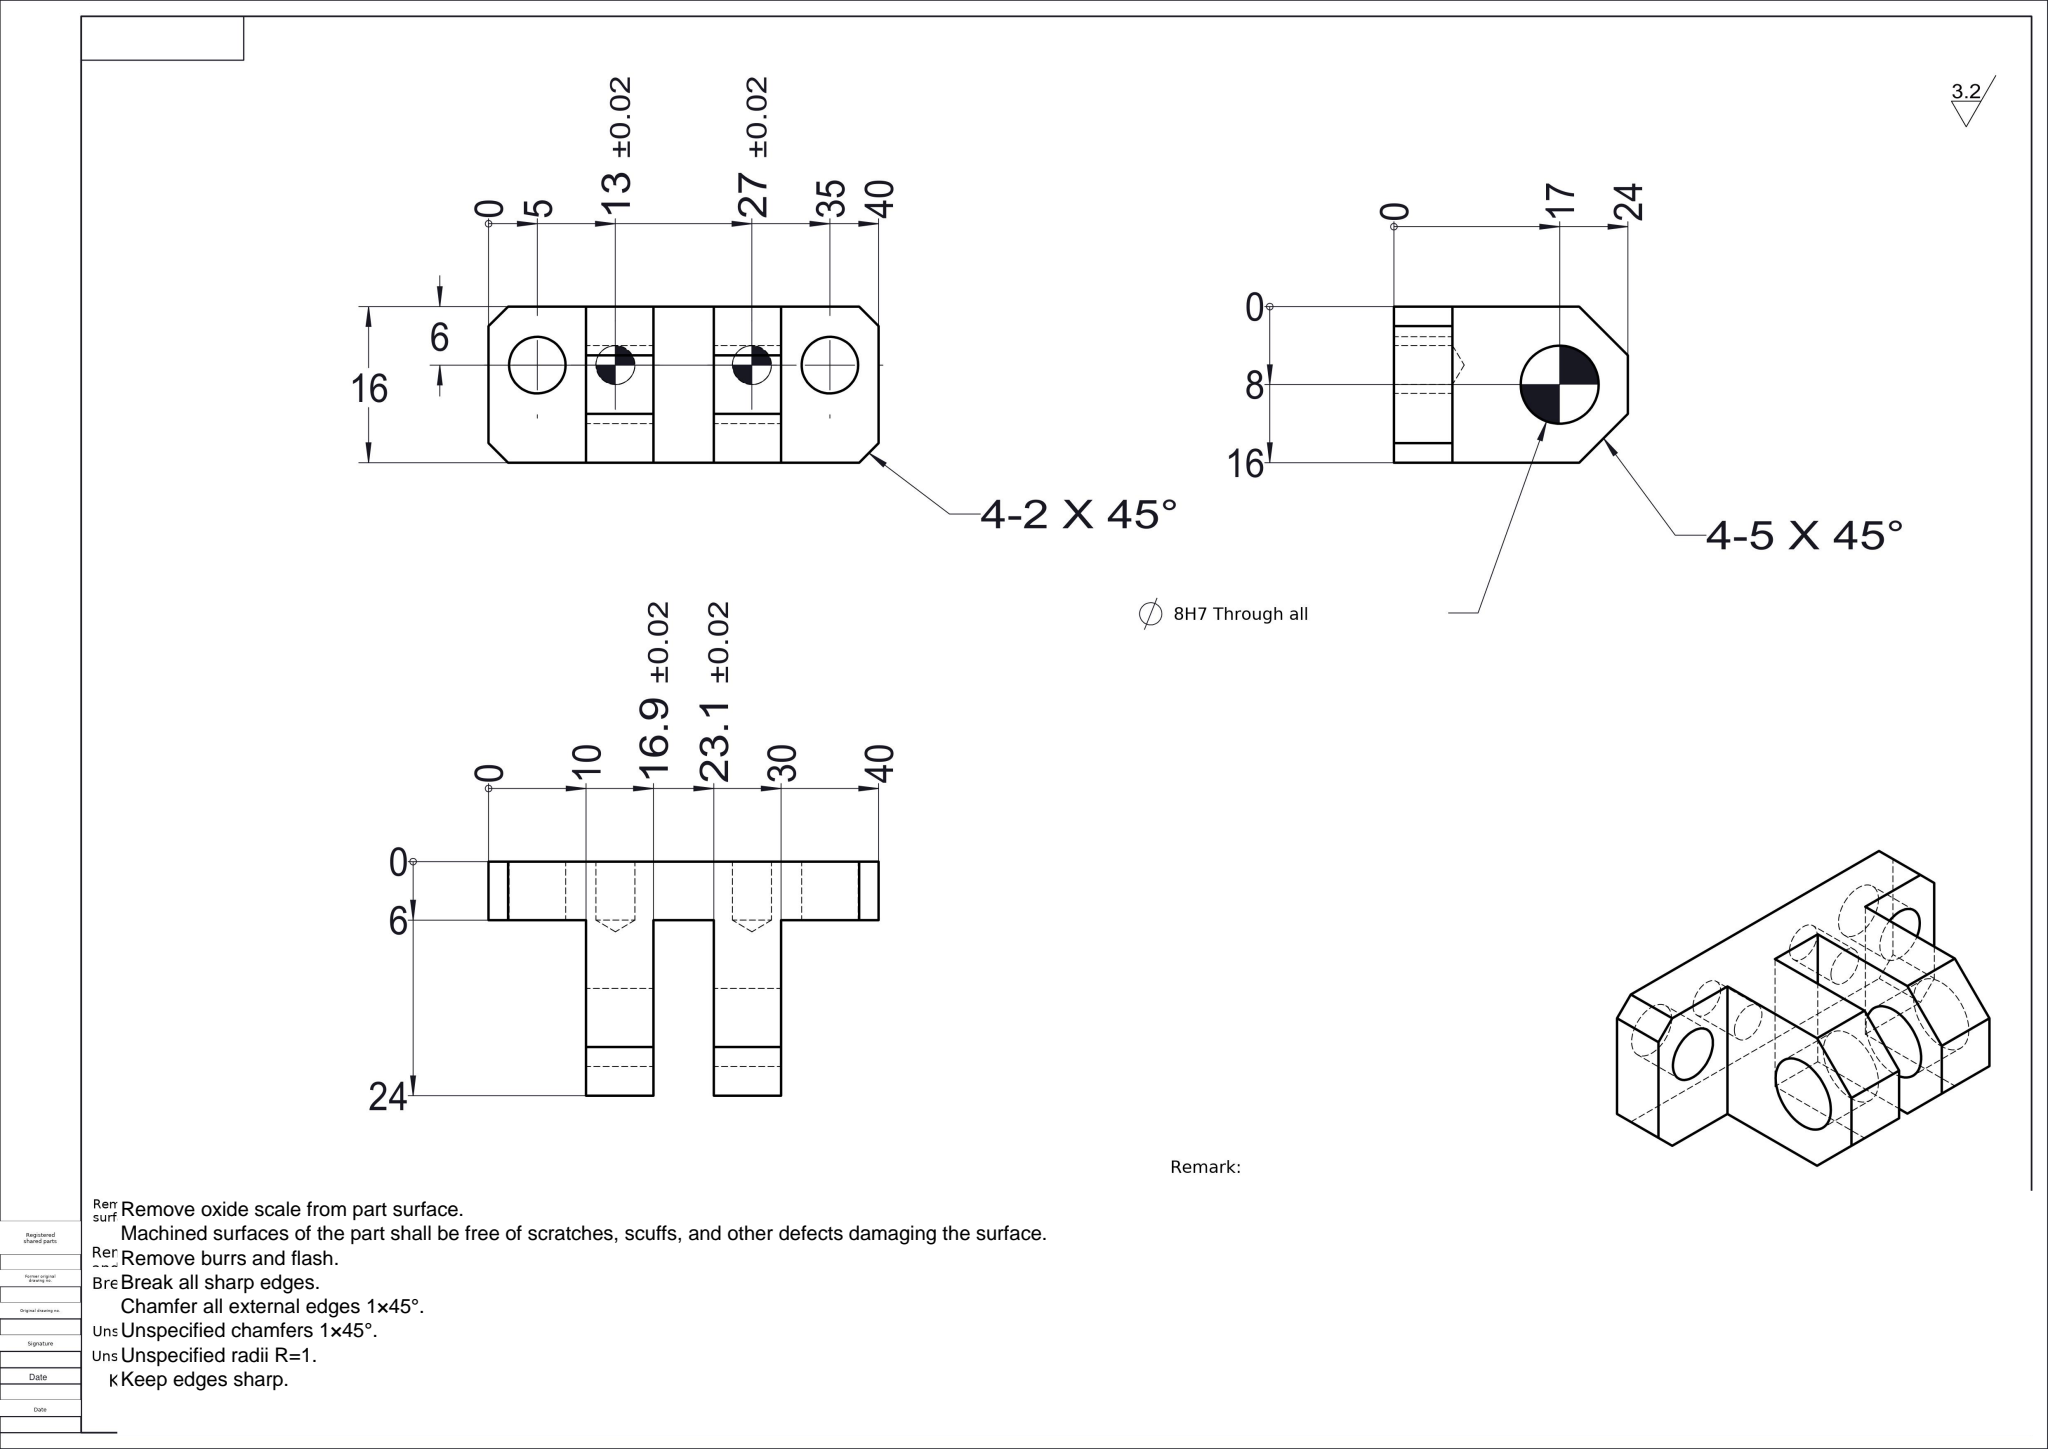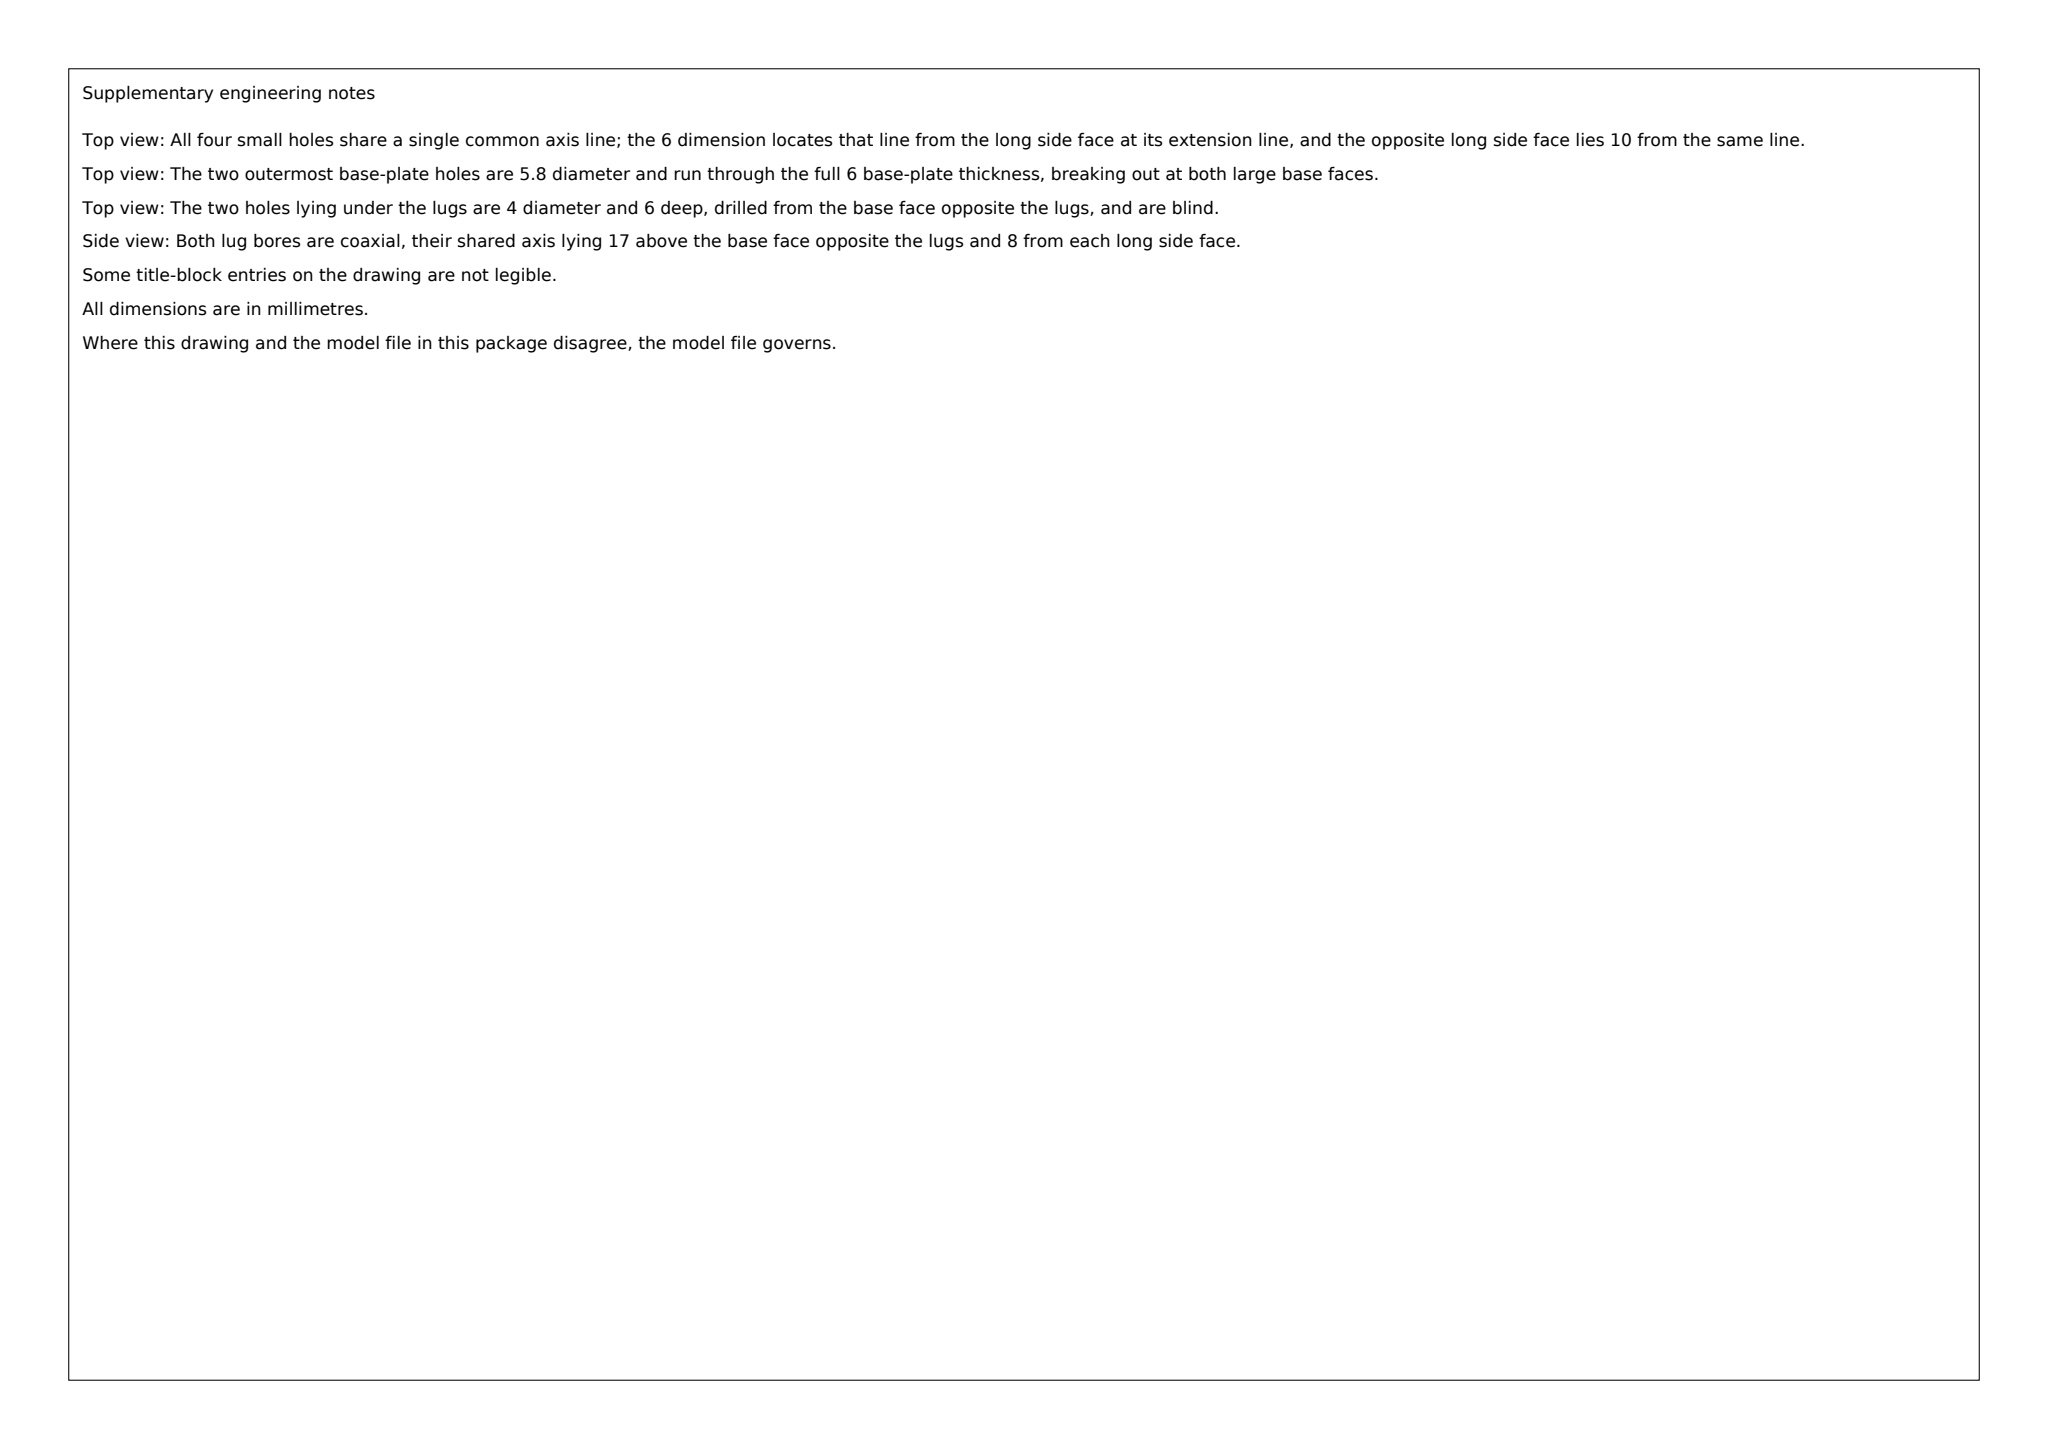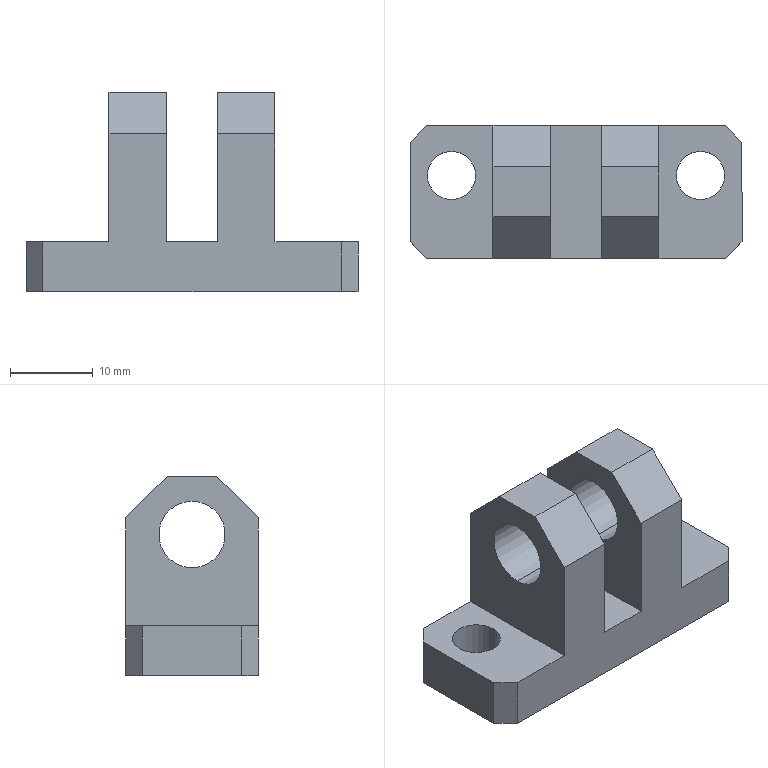Part | SolidWorks | mm | 1 solid | 38 faces | box 40 x 16 x 24 mm | volume 6250 mm3 | plane 22 | cylinder 12 | cone 4 | commonest cylinder face diameters 4 x4 5.8 x4 8 x4
Drawing notes:
2X Ø4 VERT HOLE AT 13 & 27 FROM LH END, TOP VIEW | from the solid: cylinders dia 4.0 axis z at (x=13,y=10) and (x=27,y=10)
2X Ø4 DP 6 FULL DIA + 118° DRILL PT FROM TOP FACE | from the solid: dia 4.0 z-cyl length 6.0; cones 118.0 included angle, ref dia 4.0 (4 off)
2X Ø5.8 VERT HOLE AT 5 & 35 FROM LH END, TOP VIEW | from the solid: cylinders dia 5.8 axis z at (x=5,y=10) and (x=35,y=10)
2X Ø5.8 THRU 6 THK PLATE, FLAT BOTTOM, NO DRILL PT | from the solid: dia 5.8 z-cyl length 6.0 = plate thk (z planes 0 and 6); no cone at ref dia 5.8
build123d program:
from build123d import *

# Parameters (mm, degrees)
SKETCH1_W                      = 40
SKETCH1_H                      = 16
BOSS_EXTRUDE1_DEPTH            = 6
SKETCH2_W                      = 6.9
SKETCH2_H                      = 16
BOSS_EXTRUDE2_DEPTH            = 18
CHAMFER1_SIZE                  = 5
SIZE_MM_DOWEL_PIN_HOLE_1_D     = 8
CHAMFER2_SIZE                  = 2
F_5_8_5_8_DIAMETER_HOLE1_D     = 5.8
SIZE_MM_DOWEL_PIN_HOLE_2_D     = 4
SIZE_MM_DOWEL_PIN_HOLE_2_DEPTH = 6
SIZE_MM_DOWEL_PIN_HOLE_2_TIP   = 1.202


with BuildPart() as part:
    # Sketch1 → Boss-Extrude1 (new body)
    with BuildSketch(Plane.XY):
        Rectangle(SKETCH1_W, SKETCH1_H)
    extrude(amount=BOSS_EXTRUDE1_DEPTH)

    # Sketch2 → Boss-Extrude2 (add)
    with BuildSketch(Plane.XY.offset(6)):
        with Locations((-6.55, 0)):
            Rectangle(SKETCH2_W, SKETCH2_H)
        with Locations((6.55, 0)):
            Rectangle(SKETCH2_W, SKETCH2_H)
    extrude(amount=BOSS_EXTRUDE2_DEPTH)

    # Chamfer1
    chamfer1_edges = [part.edges().sort_by_distance(p)[0] for p in [
        (-6.55, -8, 24),
        (-6.55, 8, 24),
        (6.55, -8, 24),
        (6.55, 8, 24),
    ]]
    chamfer(chamfer1_edges, length=CHAMFER1_SIZE)

    # Size mm Dowel Pin Hole 1 (through all)
    with Locations(Plane.ZY.offset(10)):
        with Locations((17, 0)):
            Hole(SIZE_MM_DOWEL_PIN_HOLE_1_D / 2)

    # Chamfer2
    chamfer2_edges = [part.edges().sort_by_distance(p)[0] for p in [
        (20, -8, 3),
        (-20, -8, 3),
        (-20, 8, 3),
        (20, 8, 3),
    ]]
    chamfer(chamfer2_edges, length=CHAMFER2_SIZE)

    # 5.8 _5.8_ Diameter Hole1 (through all)
    with Locations(Plane.XY.offset(6)):
        with Locations((-15, 2), (15, 2)):
            Hole(F_5_8_5_8_DIAMETER_HOLE1_D / 2)

    # Size mm Dowel Pin Hole 2
    with Locations(Plane(origin=(0, 0, 0), x_dir=(-1, 0, 0), z_dir=(0, 0, -1))):
        with Locations((7, 2), (-7, 2)):
            Hole(SIZE_MM_DOWEL_PIN_HOLE_2_D / 2, depth=SIZE_MM_DOWEL_PIN_HOLE_2_DEPTH)
            with Locations((0, 0, -(SIZE_MM_DOWEL_PIN_HOLE_2_DEPTH + SIZE_MM_DOWEL_PIN_HOLE_2_TIP / 2))):  # 118° drill point
                Cone(0, SIZE_MM_DOWEL_PIN_HOLE_2_D / 2, SIZE_MM_DOWEL_PIN_HOLE_2_TIP, mode=Mode.SUBTRACT)


solid = part.part